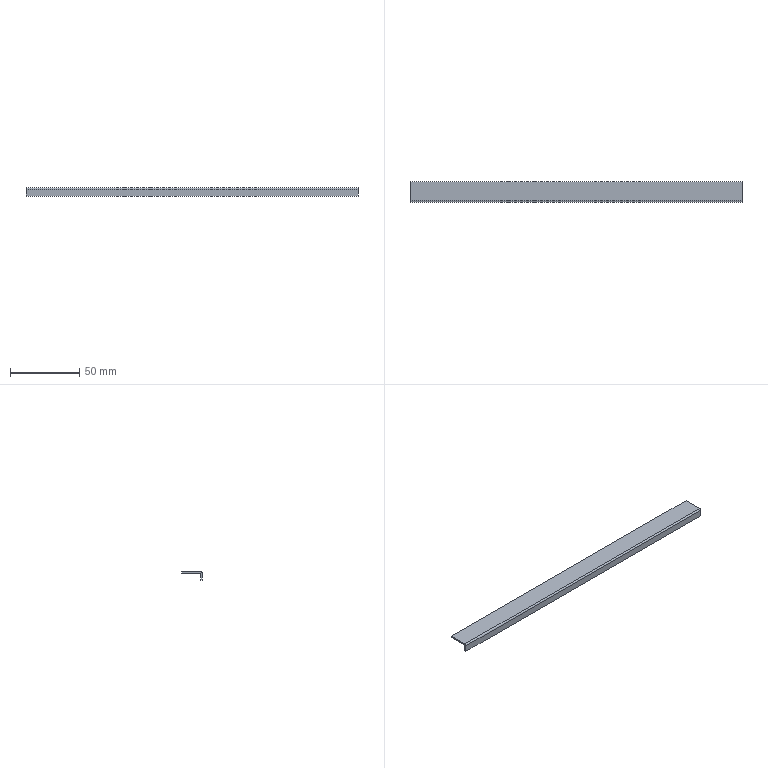Component | SolidWorks | Lampshade-1_Lampshade3-1 | 1 solid | 14 faces | box 240 x 15 x 6 mm | volume 4738 mm3 | plane 12 | cylinder 2 | commonest cylinder face diameters 0.2 x1 2.2 x1
STEP:
#1=CARTESIAN_POINT('',(3.372,-3.543,5.965));
#2=VERTEX_POINT('',#1);
#3=CARTESIAN_POINT('',(3.372,-3.543,5.925));
#4=VERTEX_POINT('',#3);
#5=CARTESIAN_POINT('',(3.372,-3.543,5.965));
#6=DIRECTION('',(0.,-0.,-1.));
#7=VECTOR('',#6,39.37);
#8=LINE('',#5,#7);
#9=EDGE_CURVE('',#2,#4,#8,.T.);
#10=ORIENTED_EDGE('',*,*,#9,.F.);
#11=CARTESIAN_POINT('',(3.372,-3.586,5.921));
#12=VERTEX_POINT('',#11);
#13=CARTESIAN_POINT('',(3.372,-3.543,5.921));
#14=DIRECTION('',(1.,-0.,0.));
#15=DIRECTION('',(0.,0.,1.));
#16=AXIS2_PLACEMENT_3D('',#13,#14,#15);
#17=CIRCLE('',#16,0.04331);
#18=EDGE_CURVE('',#2,#12,#17,.T.);
#19=ORIENTED_EDGE('',*,*,#18,.T.);
#20=CARTESIAN_POINT('',(3.372,-3.547,5.921));
#21=VERTEX_POINT('',#20);
#22=CARTESIAN_POINT('',(3.372,-3.547,5.921));
#23=DIRECTION('',(-0.,-1.,0.));
#24=VECTOR('',#23,39.37);
#25=LINE('',#22,#24);
#26=EDGE_CURVE('',#21,#12,#25,.T.);
#27=ORIENTED_EDGE('',*,*,#26,.F.);
#28=CARTESIAN_POINT('',(3.372,-3.543,5.921));
#29=DIRECTION('',(1.,-0.,0.));
#30=DIRECTION('',(0.,0.,-1.));
#31=AXIS2_PLACEMENT_3D('',#28,#29,#30);
#32=CIRCLE('',#31,0.003937);
#33=EDGE_CURVE('',#4,#21,#32,.T.);
#34=ORIENTED_EDGE('',*,*,#33,.F.);
#35=EDGE_LOOP('',(#10,#19,#27,#34));
#36=FACE_OUTER_BOUND('',#35,.T.);
#37=CARTESIAN_POINT('',(3.372,-3.543,5.965));
#38=DIRECTION('',(1.,-0.,0.));
#39=DIRECTION('',(0.,-0.,-1.));
#40=AXIS2_PLACEMENT_3D('',#37,#38,#39);
#41=PLANE('',#40);
#42=ADVANCED_FACE('',(#36),#41,.T.);
#43=CARTESIAN_POINT('',(3.372,-2.996,5.965));
#44=VERTEX_POINT('',#43);
#45=CARTESIAN_POINT('',(3.372,-2.996,5.965));
#46=DIRECTION('',(-0.,-1.,0.));
#47=VECTOR('',#46,39.37);
#48=LINE('',#45,#47);
#49=EDGE_CURVE('',#44,#2,#48,.T.);
#50=ORIENTED_EDGE('',*,*,#49,.T.);
#51=ORIENTED_EDGE('',*,*,#9,.T.);
#52=CARTESIAN_POINT('',(3.372,-2.996,5.925));
#53=VERTEX_POINT('',#52);
#54=CARTESIAN_POINT('',(3.372,-2.996,5.925));
#55=DIRECTION('',(-0.,-1.,0.));
#56=VECTOR('',#55,39.37);
#57=LINE('',#54,#56);
#58=EDGE_CURVE('',#53,#4,#57,.T.);
#59=ORIENTED_EDGE('',*,*,#58,.F.);
#60=CARTESIAN_POINT('',(3.372,-2.996,5.965));
#61=DIRECTION('',(0.,-0.,-1.));
#62=VECTOR('',#61,39.37);
#63=LINE('',#60,#62);
#64=EDGE_CURVE('',#44,#53,#63,.T.);
#65=ORIENTED_EDGE('',*,*,#64,.F.);
#66=EDGE_LOOP('',(#50,#51,#59,#65));
#67=FACE_OUTER_BOUND('',#66,.T.);
#68=CARTESIAN_POINT('',(3.372,-3.547,5.921));
#69=DIRECTION('',(1.,-0.,0.));
#70=DIRECTION('',(0.,-0.,-1.));
#71=AXIS2_PLACEMENT_3D('',#68,#69,#70);
#72=PLANE('',#71);
#73=ADVANCED_FACE('',(#67),#72,.T.);
#74=CARTESIAN_POINT('',(-6.077,-3.586,5.921));
#75=VERTEX_POINT('',#74);
#76=CARTESIAN_POINT('',(-6.077,-3.547,5.921));
#77=VERTEX_POINT('',#76);
#78=CARTESIAN_POINT('',(-6.077,-3.586,5.921));
#79=DIRECTION('',(0.,1.,-0.));
#80=VECTOR('',#79,39.37);
#81=LINE('',#78,#80);
#82=EDGE_CURVE('',#75,#77,#81,.T.);
#83=ORIENTED_EDGE('',*,*,#82,.F.);
#84=CARTESIAN_POINT('',(-6.077,-3.543,5.965));
#85=VERTEX_POINT('',#84);
#86=CARTESIAN_POINT('',(-6.077,-3.543,5.921));
#87=DIRECTION('',(1.,-0.,0.));
#88=DIRECTION('',(0.,0.,1.));
#89=AXIS2_PLACEMENT_3D('',#86,#87,#88);
#90=CIRCLE('',#89,0.04331);
#91=EDGE_CURVE('',#85,#75,#90,.T.);
#92=ORIENTED_EDGE('',*,*,#91,.F.);
#93=CARTESIAN_POINT('',(-6.077,-3.543,5.925));
#94=VERTEX_POINT('',#93);
#95=CARTESIAN_POINT('',(-6.077,-3.543,5.925));
#96=DIRECTION('',(0.,0.,1.));
#97=VECTOR('',#96,39.37);
#98=LINE('',#95,#97);
#99=EDGE_CURVE('',#94,#85,#98,.T.);
#100=ORIENTED_EDGE('',*,*,#99,.F.);
#101=CARTESIAN_POINT('',(-6.077,-3.543,5.921));
#102=DIRECTION('',(1.,-0.,0.));
#103=DIRECTION('',(0.,0.,-1.));
#104=AXIS2_PLACEMENT_3D('',#101,#102,#103);
#105=CIRCLE('',#104,0.003937);
#106=EDGE_CURVE('',#94,#77,#105,.T.);
#107=ORIENTED_EDGE('',*,*,#106,.T.);
#108=EDGE_LOOP('',(#83,#92,#100,#107));
#109=FACE_OUTER_BOUND('',#108,.T.);
#110=CARTESIAN_POINT('',(-6.077,-3.586,5.921));
#111=DIRECTION('',(-1.,0.,-0.));
#112=DIRECTION('',(0.,0.,1.));
#113=AXIS2_PLACEMENT_3D('',#110,#111,#112);
#114=PLANE('',#113);
#115=ADVANCED_FACE('',(#109),#114,.T.);
#116=CARTESIAN_POINT('',(-6.077,-3.586,5.728));
#117=VERTEX_POINT('',#116);
#118=CARTESIAN_POINT('',(-6.077,-3.586,5.965));
#119=DIRECTION('',(0.,-0.,-1.));
#120=VECTOR('',#119,39.37);
#121=LINE('',#118,#120);
#122=EDGE_CURVE('',#75,#117,#121,.T.);
#123=ORIENTED_EDGE('',*,*,#122,.F.);
#124=ORIENTED_EDGE('',*,*,#82,.T.);
#125=CARTESIAN_POINT('',(-6.077,-3.547,5.728));
#126=VERTEX_POINT('',#125);
#127=CARTESIAN_POINT('',(-6.077,-3.547,5.965));
#128=DIRECTION('',(0.,-0.,-1.));
#129=VECTOR('',#128,39.37);
#130=LINE('',#127,#129);
#131=EDGE_CURVE('',#77,#126,#130,.T.);
#132=ORIENTED_EDGE('',*,*,#131,.T.);
#133=CARTESIAN_POINT('',(-6.077,-3.547,5.728));
#134=DIRECTION('',(-0.,-1.,0.));
#135=VECTOR('',#134,39.37);
#136=LINE('',#133,#135);
#137=EDGE_CURVE('',#126,#117,#136,.T.);
#138=ORIENTED_EDGE('',*,*,#137,.T.);
#139=EDGE_LOOP('',(#123,#124,#132,#138));
#140=FACE_OUTER_BOUND('',#139,.T.);
#141=CARTESIAN_POINT('',(-6.077,-3.543,5.925));
#142=DIRECTION('',(-1.,0.,-0.));
#143=DIRECTION('',(0.,0.,1.));
#144=AXIS2_PLACEMENT_3D('',#141,#142,#143);
#145=PLANE('',#144);
#146=ADVANCED_FACE('',(#140),#145,.T.);
#147=ORIENTED_EDGE('',*,*,#122,.T.);
#148=CARTESIAN_POINT('',(3.372,-3.586,5.728));
#149=VERTEX_POINT('',#148);
#150=CARTESIAN_POINT('',(3.372,-3.586,5.728));
#151=DIRECTION('',(-1.,0.,0.));
#152=VECTOR('',#151,39.37);
#153=LINE('',#150,#152);
#154=EDGE_CURVE('',#149,#117,#153,.T.);
#155=ORIENTED_EDGE('',*,*,#154,.F.);
#156=CARTESIAN_POINT('',(3.372,-3.586,5.965));
#157=DIRECTION('',(0.,-0.,-1.));
#158=VECTOR('',#157,39.37);
#159=LINE('',#156,#158);
#160=EDGE_CURVE('',#12,#149,#159,.T.);
#161=ORIENTED_EDGE('',*,*,#160,.F.);
#162=CARTESIAN_POINT('',(3.372,-3.586,5.921));
#163=DIRECTION('',(-1.,0.,0.));
#164=VECTOR('',#163,39.37);
#165=LINE('',#162,#164);
#166=EDGE_CURVE('',#12,#75,#165,.T.);
#167=ORIENTED_EDGE('',*,*,#166,.T.);
#168=EDGE_LOOP('',(#147,#155,#161,#167));
#169=FACE_OUTER_BOUND('',#168,.T.);
#170=CARTESIAN_POINT('',(3.372,-3.586,5.965));
#171=DIRECTION('',(0.,1.,-0.));
#172=DIRECTION('',(1.,-0.,0.));
#173=AXIS2_PLACEMENT_3D('',#170,#171,#172);
#174=PLANE('',#173);
#175=ADVANCED_FACE('',(#169),#174,.F.);
#176=ORIENTED_EDGE('',*,*,#137,.F.);
#177=CARTESIAN_POINT('',(3.372,-3.547,5.728));
#178=VERTEX_POINT('',#177);
#179=CARTESIAN_POINT('',(3.372,-3.547,5.728));
#180=DIRECTION('',(-1.,0.,0.));
#181=VECTOR('',#180,39.37);
#182=LINE('',#179,#181);
#183=EDGE_CURVE('',#178,#126,#182,.T.);
#184=ORIENTED_EDGE('',*,*,#183,.F.);
#185=CARTESIAN_POINT('',(3.372,-3.547,5.728));
#186=DIRECTION('',(-0.,-1.,0.));
#187=VECTOR('',#186,39.37);
#188=LINE('',#185,#187);
#189=EDGE_CURVE('',#178,#149,#188,.T.);
#190=ORIENTED_EDGE('',*,*,#189,.T.);
#191=ORIENTED_EDGE('',*,*,#154,.T.);
#192=EDGE_LOOP('',(#176,#184,#190,#191));
#193=FACE_OUTER_BOUND('',#192,.T.);
#194=CARTESIAN_POINT('',(3.372,-3.547,5.728));
#195=DIRECTION('',(-0.,-0.,-1.));
#196=DIRECTION('',(-1.,0.,0.));
#197=AXIS2_PLACEMENT_3D('',#194,#195,#196);
#198=PLANE('',#197);
#199=ADVANCED_FACE('',(#193),#198,.T.);
#200=ORIENTED_EDGE('',*,*,#131,.F.);
#201=CARTESIAN_POINT('',(3.372,-3.547,5.921));
#202=DIRECTION('',(-1.,0.,0.));
#203=VECTOR('',#202,39.37);
#204=LINE('',#201,#203);
#205=EDGE_CURVE('',#21,#77,#204,.T.);
#206=ORIENTED_EDGE('',*,*,#205,.F.);
#207=CARTESIAN_POINT('',(3.372,-3.547,5.965));
#208=DIRECTION('',(0.,-0.,-1.));
#209=VECTOR('',#208,39.37);
#210=LINE('',#207,#209);
#211=EDGE_CURVE('',#21,#178,#210,.T.);
#212=ORIENTED_EDGE('',*,*,#211,.T.);
#213=ORIENTED_EDGE('',*,*,#183,.T.);
#214=EDGE_LOOP('',(#200,#206,#212,#213));
#215=FACE_OUTER_BOUND('',#214,.T.);
#216=CARTESIAN_POINT('',(3.372,-3.547,5.965));
#217=DIRECTION('',(0.,1.,-0.));
#218=DIRECTION('',(1.,-0.,0.));
#219=AXIS2_PLACEMENT_3D('',#216,#217,#218);
#220=PLANE('',#219);
#221=ADVANCED_FACE('',(#215),#220,.T.);
#222=ORIENTED_EDGE('',*,*,#106,.F.);
#223=CARTESIAN_POINT('',(3.372,-3.543,5.925));
#224=DIRECTION('',(-1.,0.,0.));
#225=VECTOR('',#224,39.37);
#226=LINE('',#223,#225);
#227=EDGE_CURVE('',#4,#94,#226,.T.);
#228=ORIENTED_EDGE('',*,*,#227,.F.);
#229=ORIENTED_EDGE('',*,*,#33,.T.);
#230=ORIENTED_EDGE('',*,*,#205,.T.);
#231=EDGE_LOOP('',(#222,#228,#229,#230));
#232=FACE_OUTER_BOUND('',#231,.T.);
#233=CARTESIAN_POINT('',(3.372,-3.543,5.921));
#234=DIRECTION('',(-1.,0.,0.));
#235=DIRECTION('',(0.,0.,1.));
#236=AXIS2_PLACEMENT_3D('',#233,#234,#235);
#237=CYLINDRICAL_SURFACE('',#236,0.003937);
#238=ADVANCED_FACE('',(#232),#237,.F.);
#239=CARTESIAN_POINT('',(-6.077,-2.996,5.925));
#240=VERTEX_POINT('',#239);
#241=CARTESIAN_POINT('',(-6.077,-2.996,5.925));
#242=DIRECTION('',(-0.,-1.,0.));
#243=VECTOR('',#242,39.37);
#244=LINE('',#241,#243);
#245=EDGE_CURVE('',#240,#94,#244,.T.);
#246=ORIENTED_EDGE('',*,*,#245,.F.);
#247=CARTESIAN_POINT('',(3.372,-2.996,5.925));
#248=DIRECTION('',(-1.,0.,0.));
#249=VECTOR('',#248,39.37);
#250=LINE('',#247,#249);
#251=EDGE_CURVE('',#53,#240,#250,.T.);
#252=ORIENTED_EDGE('',*,*,#251,.F.);
#253=ORIENTED_EDGE('',*,*,#58,.T.);
#254=ORIENTED_EDGE('',*,*,#227,.T.);
#255=EDGE_LOOP('',(#246,#252,#253,#254));
#256=FACE_OUTER_BOUND('',#255,.T.);
#257=CARTESIAN_POINT('',(3.372,-2.996,5.925));
#258=DIRECTION('',(-0.,-0.,-1.));
#259=DIRECTION('',(-1.,0.,0.));
#260=AXIS2_PLACEMENT_3D('',#257,#258,#259);
#261=PLANE('',#260);
#262=ADVANCED_FACE('',(#256),#261,.T.);
#263=CARTESIAN_POINT('',(-6.077,-2.996,5.965));
#264=VERTEX_POINT('',#263);
#265=CARTESIAN_POINT('',(-6.077,-2.996,5.965));
#266=DIRECTION('',(0.,-0.,-1.));
#267=VECTOR('',#266,39.37);
#268=LINE('',#265,#267);
#269=EDGE_CURVE('',#264,#240,#268,.T.);
#270=ORIENTED_EDGE('',*,*,#269,.F.);
#271=CARTESIAN_POINT('',(3.372,-2.996,5.965));
#272=DIRECTION('',(-1.,0.,0.));
#273=VECTOR('',#272,39.37);
#274=LINE('',#271,#273);
#275=EDGE_CURVE('',#44,#264,#274,.T.);
#276=ORIENTED_EDGE('',*,*,#275,.F.);
#277=ORIENTED_EDGE('',*,*,#64,.T.);
#278=ORIENTED_EDGE('',*,*,#251,.T.);
#279=EDGE_LOOP('',(#270,#276,#277,#278));
#280=FACE_OUTER_BOUND('',#279,.T.);
#281=CARTESIAN_POINT('',(3.372,-2.996,5.965));
#282=DIRECTION('',(0.,1.,-0.));
#283=DIRECTION('',(1.,-0.,0.));
#284=AXIS2_PLACEMENT_3D('',#281,#282,#283);
#285=PLANE('',#284);
#286=ADVANCED_FACE('',(#280),#285,.T.);
#287=CARTESIAN_POINT('',(-6.077,-2.996,5.965));
#288=DIRECTION('',(-0.,-1.,0.));
#289=VECTOR('',#288,39.37);
#290=LINE('',#287,#289);
#291=EDGE_CURVE('',#264,#85,#290,.T.);
#292=ORIENTED_EDGE('',*,*,#291,.T.);
#293=CARTESIAN_POINT('',(3.372,-3.543,5.965));
#294=DIRECTION('',(-1.,0.,0.));
#295=VECTOR('',#294,39.37);
#296=LINE('',#293,#295);
#297=EDGE_CURVE('',#2,#85,#296,.T.);
#298=ORIENTED_EDGE('',*,*,#297,.F.);
#299=ORIENTED_EDGE('',*,*,#49,.F.);
#300=ORIENTED_EDGE('',*,*,#275,.T.);
#301=EDGE_LOOP('',(#292,#298,#299,#300));
#302=FACE_OUTER_BOUND('',#301,.T.);
#303=CARTESIAN_POINT('',(3.372,-2.996,5.965));
#304=DIRECTION('',(-0.,-0.,-1.));
#305=DIRECTION('',(-1.,0.,0.));
#306=AXIS2_PLACEMENT_3D('',#303,#304,#305);
#307=PLANE('',#306);
#308=ADVANCED_FACE('',(#302),#307,.F.);
#309=ORIENTED_EDGE('',*,*,#91,.T.);
#310=ORIENTED_EDGE('',*,*,#166,.F.);
#311=ORIENTED_EDGE('',*,*,#18,.F.);
#312=ORIENTED_EDGE('',*,*,#297,.T.);
#313=EDGE_LOOP('',(#309,#310,#311,#312));
#314=FACE_OUTER_BOUND('',#313,.T.);
#315=CARTESIAN_POINT('',(3.372,-3.543,5.921));
#316=DIRECTION('',(-1.,0.,0.));
#317=DIRECTION('',(0.,0.,1.));
#318=AXIS2_PLACEMENT_3D('',#315,#316,#317);
#319=CYLINDRICAL_SURFACE('',#318,0.04331);
#320=ADVANCED_FACE('',(#314),#319,.T.);
#321=ORIENTED_EDGE('',*,*,#160,.T.);
#322=ORIENTED_EDGE('',*,*,#189,.F.);
#323=ORIENTED_EDGE('',*,*,#211,.F.);
#324=ORIENTED_EDGE('',*,*,#26,.T.);
#325=EDGE_LOOP('',(#321,#322,#323,#324));
#326=FACE_OUTER_BOUND('',#325,.T.);
#327=CARTESIAN_POINT('',(3.372,-3.543,5.921));
#328=DIRECTION('',(1.,-0.,0.));
#329=DIRECTION('',(0.,-0.,-1.));
#330=AXIS2_PLACEMENT_3D('',#327,#328,#329);
#331=PLANE('',#330);
#332=ADVANCED_FACE('',(#326),#331,.T.);
#333=ORIENTED_EDGE('',*,*,#245,.T.);
#334=ORIENTED_EDGE('',*,*,#99,.T.);
#335=ORIENTED_EDGE('',*,*,#291,.F.);
#336=ORIENTED_EDGE('',*,*,#269,.T.);
#337=EDGE_LOOP('',(#333,#334,#335,#336));
#338=FACE_OUTER_BOUND('',#337,.T.);
#339=CARTESIAN_POINT('',(-6.077,-3.543,5.921));
#340=DIRECTION('',(1.,-0.,0.));
#341=DIRECTION('',(0.,-0.,-1.));
#342=AXIS2_PLACEMENT_3D('',#339,#340,#341);
#343=PLANE('',#342);
#344=ADVANCED_FACE('',(#338),#343,.F.);
#345=CLOSED_SHELL('',(#42,#73,#115,#146,#175,#199,#221,#238,#262,#286,#308,#320,#332,#344));
#346=MANIFOLD_SOLID_BREP('',#345);
#347=CARTESIAN_POINT('',(0.,0.,0.));
#348=DIRECTION('',(0.,0.,1.));
#349=DIRECTION('',(1.,0.,0.));
#350=AXIS2_PLACEMENT_3D('',#347,#348,#349);
#351=(LENGTH_UNIT()NAMED_UNIT(*)SI_UNIT($,.METRE.));
#352=LENGTH_MEASURE_WITH_UNIT(LENGTH_MEASURE(0.0254),#351);
#353=DIMENSIONAL_EXPONENTS(1.,0.,0.,0.,0.,0.,0.);
#354=(CONVERSION_BASED_UNIT('',#352)LENGTH_UNIT()NAMED_UNIT(#353));
#355=UNCERTAINTY_MEASURE_WITH_UNIT(LENGTH_MEASURE(0.00001),#354,'','');
#356=(NAMED_UNIT(*)PLANE_ANGLE_UNIT()SI_UNIT($,.RADIAN.));
#357=(NAMED_UNIT(*)SI_UNIT($,.STERADIAN.)SOLID_ANGLE_UNIT());
#358=(GEOMETRIC_REPRESENTATION_CONTEXT(3)GLOBAL_UNCERTAINTY_ASSIGNED_CONTEXT((#355))GLOBAL_UNIT_ASSIGNED_CONTEXT((#354,#356,#357))REPRESENTATION_CONTEXT('',''));
#359=ADVANCED_BREP_SHAPE_REPRESENTATION('',(#346,#350),#358);
#360=COLOUR_RGB('',0.7922,0.8196,0.9333);
#361=FILL_AREA_STYLE_COLOUR('',#360);
#362=FILL_AREA_STYLE('',(#361));
#363=SURFACE_STYLE_FILL_AREA(#362);
#364=SURFACE_SIDE_STYLE('',(#363));
#365=SURFACE_STYLE_USAGE(.BOTH.,#364);
#366=PRESENTATION_STYLE_ASSIGNMENT((#365));
#367=STYLED_ITEM('',(#366),#346);
#368=PRESENTATION_LAYER_ASSIGNMENT('','',(#367));
#369=(LENGTH_UNIT()NAMED_UNIT(*)SI_UNIT($,.METRE.));
#370=LENGTH_MEASURE_WITH_UNIT(LENGTH_MEASURE(0.0254),#369);
#371=DIMENSIONAL_EXPONENTS(1.,0.,0.,0.,0.,0.,0.);
#372=(CONVERSION_BASED_UNIT('',#370)LENGTH_UNIT()NAMED_UNIT(#371));
#373=UNCERTAINTY_MEASURE_WITH_UNIT(LENGTH_MEASURE(0.00001),#372,'','');
#374=(NAMED_UNIT(*)PLANE_ANGLE_UNIT()SI_UNIT($,.RADIAN.));
#375=(NAMED_UNIT(*)SI_UNIT($,.STERADIAN.)SOLID_ANGLE_UNIT());
#376=(GEOMETRIC_REPRESENTATION_CONTEXT(3)GLOBAL_UNCERTAINTY_ASSIGNED_CONTEXT((#373))GLOBAL_UNIT_ASSIGNED_CONTEXT((#372,#374,#375))REPRESENTATION_CONTEXT('',''));
#377=MECHANICAL_DESIGN_GEOMETRIC_PRESENTATION_REPRESENTATION('',(#367),#376);